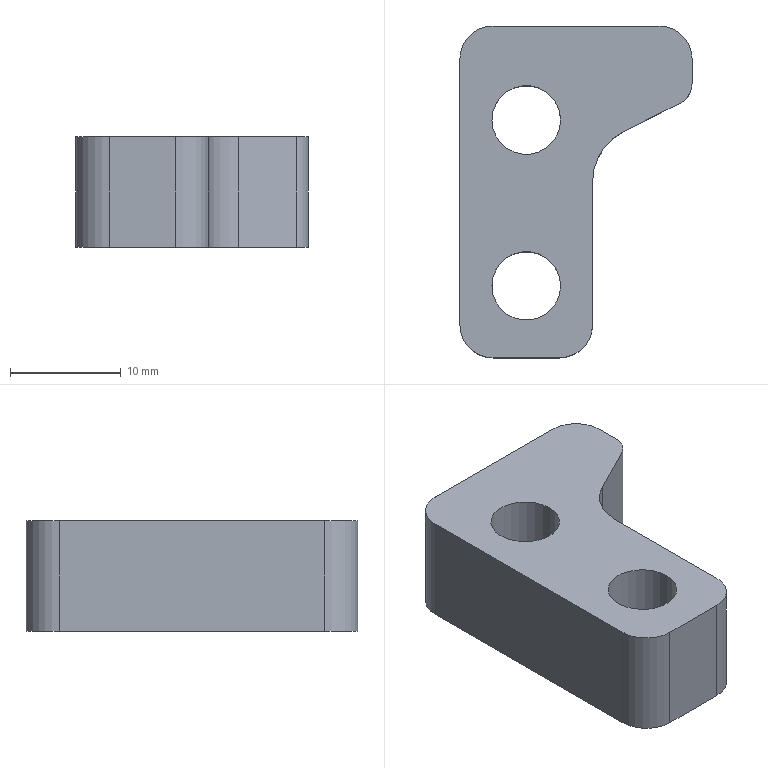CAM job | Mastercam | mm | 7 operations | part box 21 x 30 x 10
1. Facing | 23 - 63 平铣刀
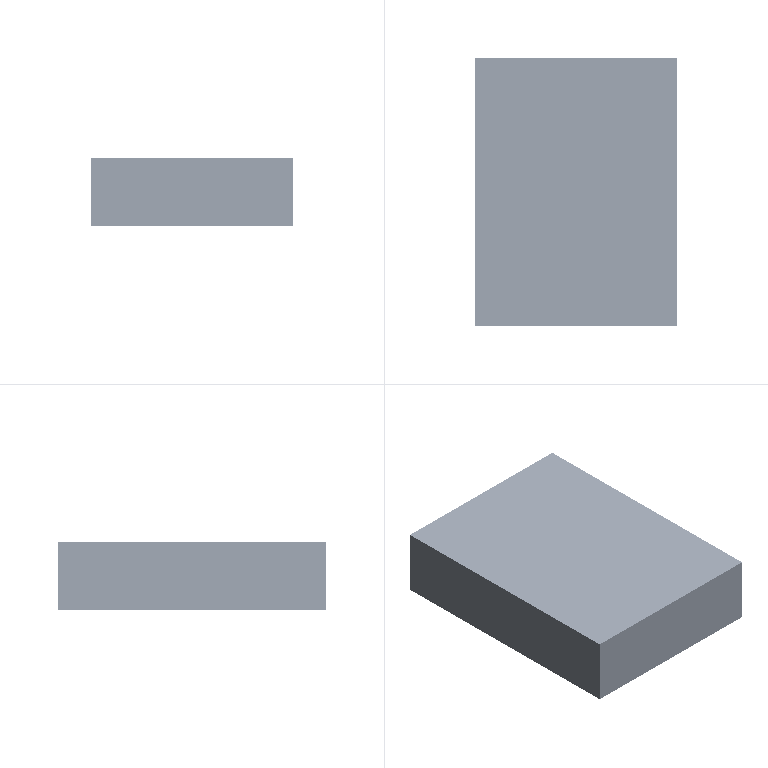2. 2D High Speed (2D Dynamic Mill) | 9 - 10 平铣刀
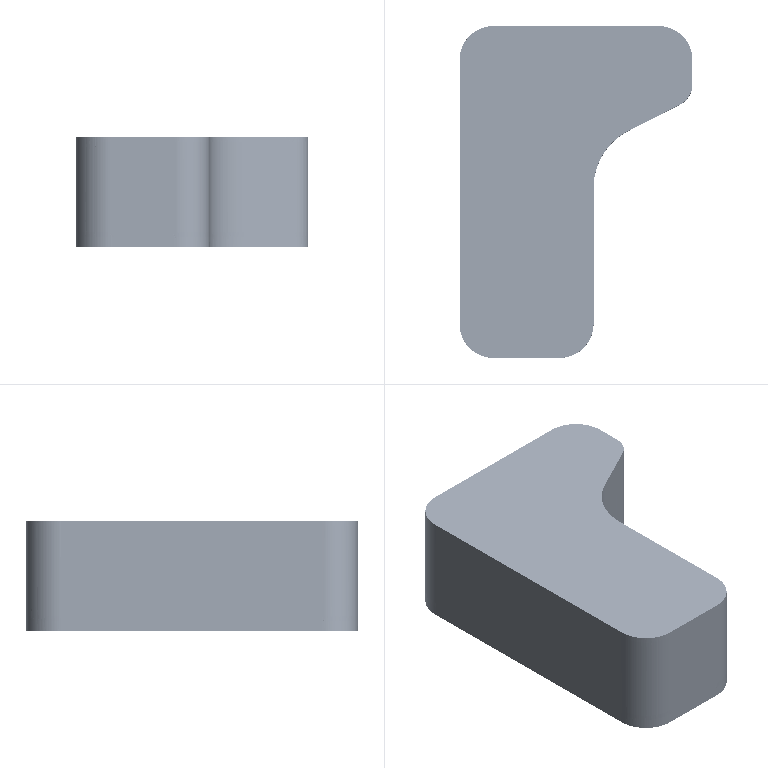3. Contour (2D) | 10 - 10 平铣刀
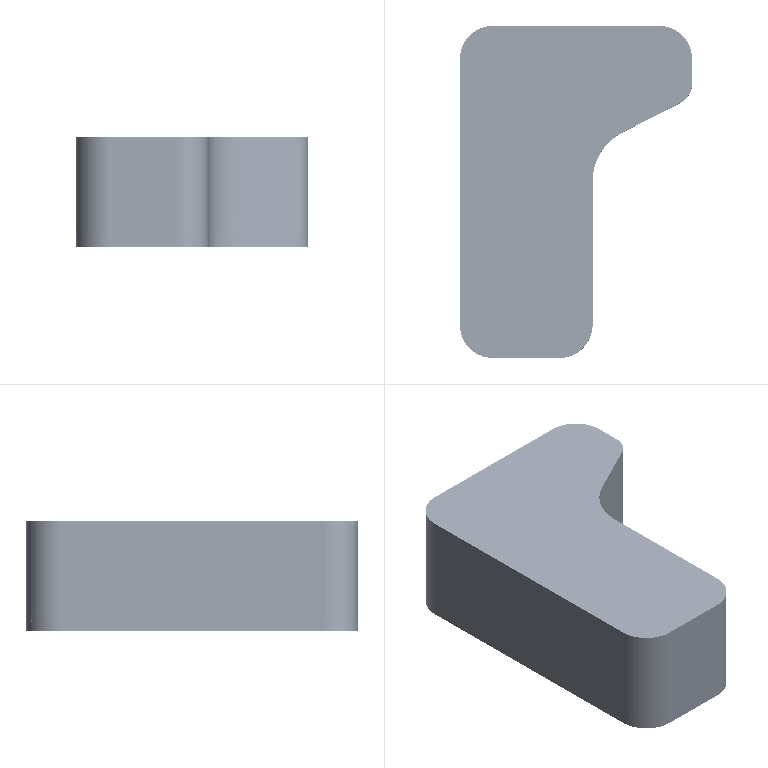4. Drill/Counterbore | 5 - 4 倒角刀
5. Contour (2D chamfer) | 5 - 4 倒角刀
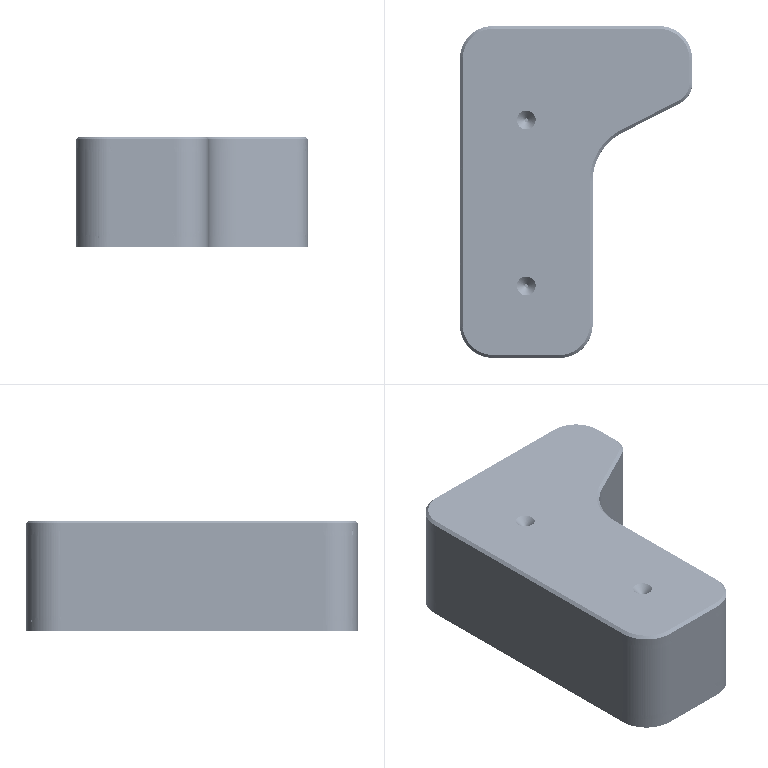6. Facing | 9 - 10 平铣刀
7. Facing | 10 - 10 平铣刀